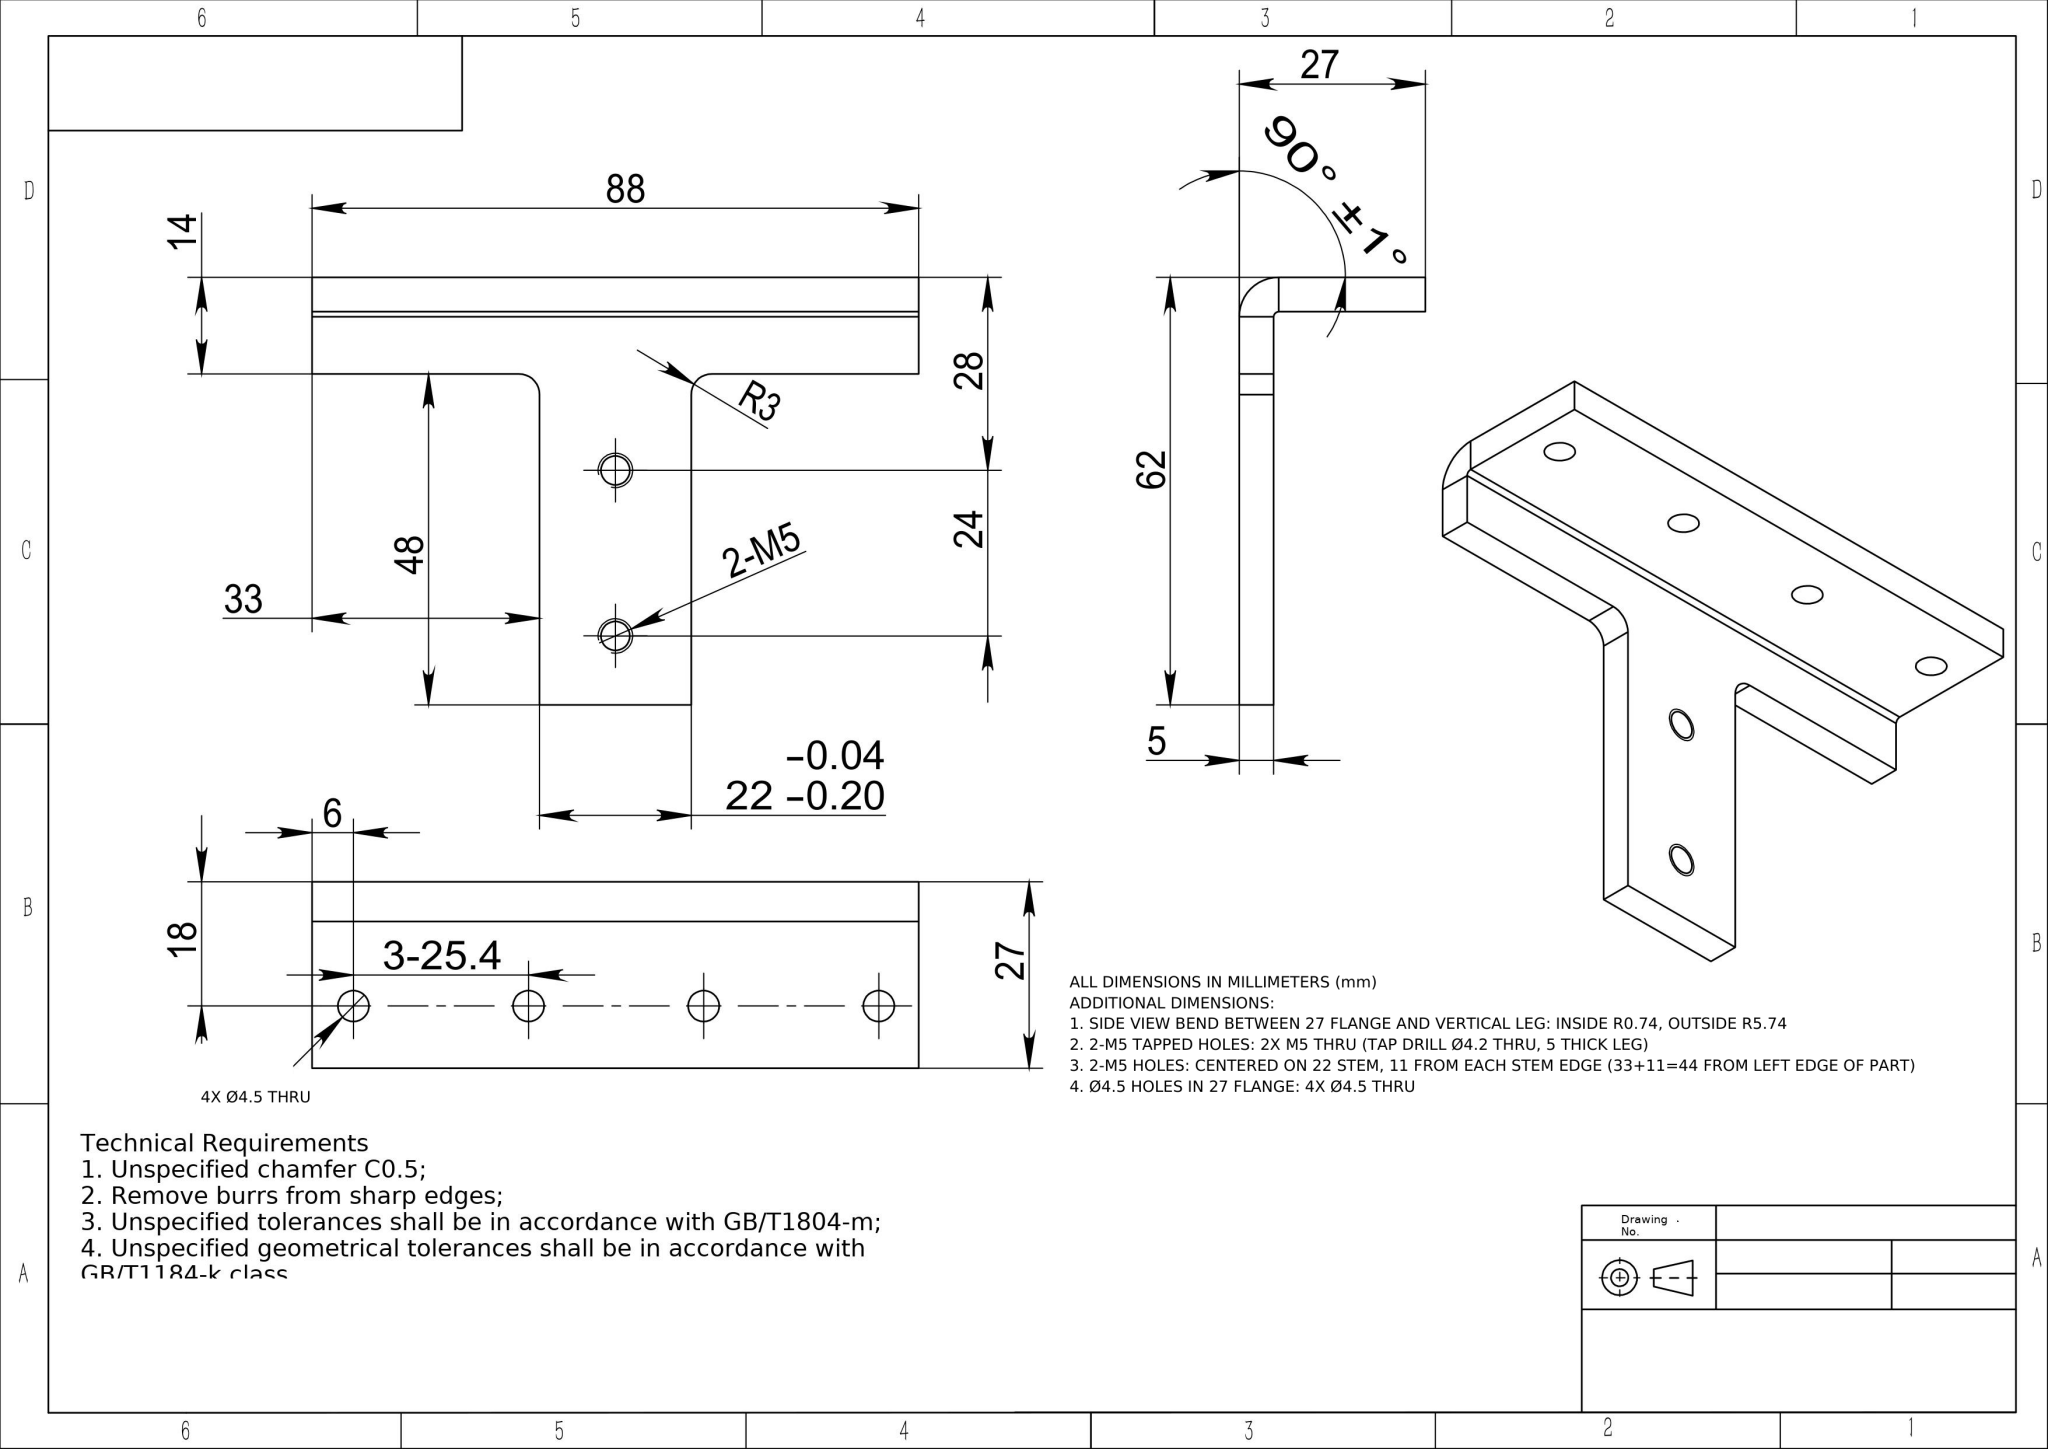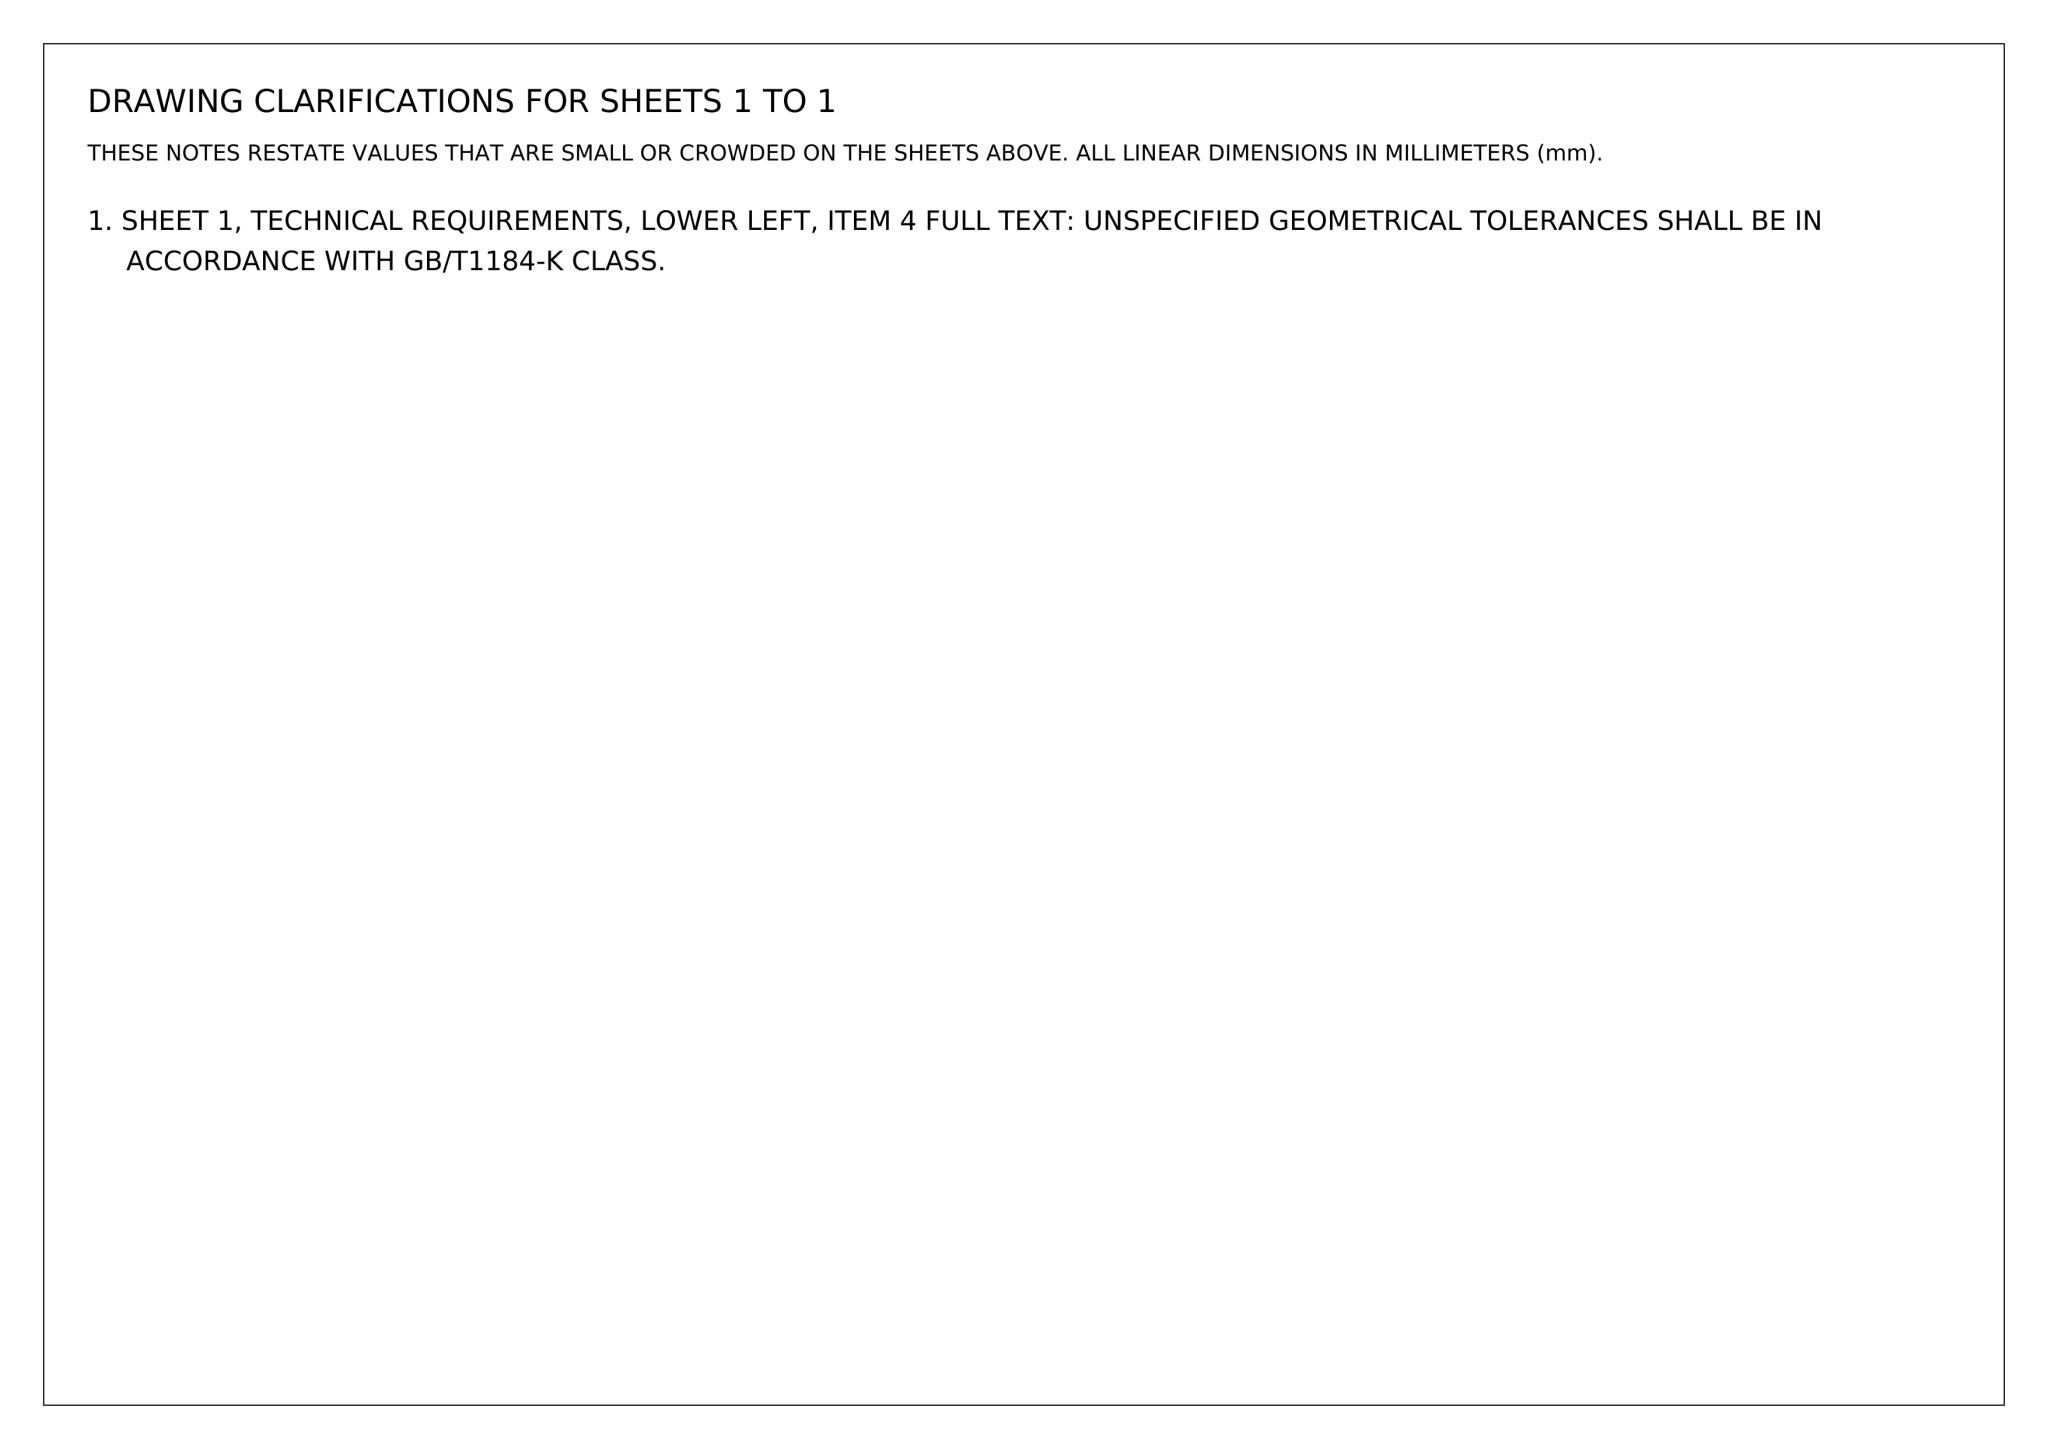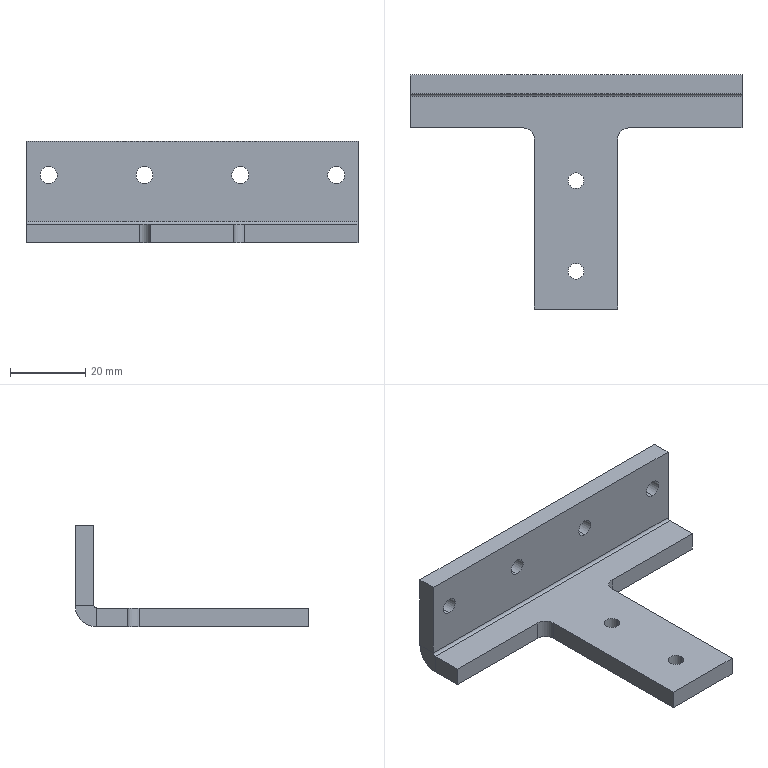Part | NX | mm | 1 solid | 32 faces | box 88 x 62 x 27 mm | volume 20071 mm3 | cylinder 16 | plane 16 | commonest cylinder face diameters 4.5 x8 4.2 x4 6 x2 11.473 x1 1.473 x1